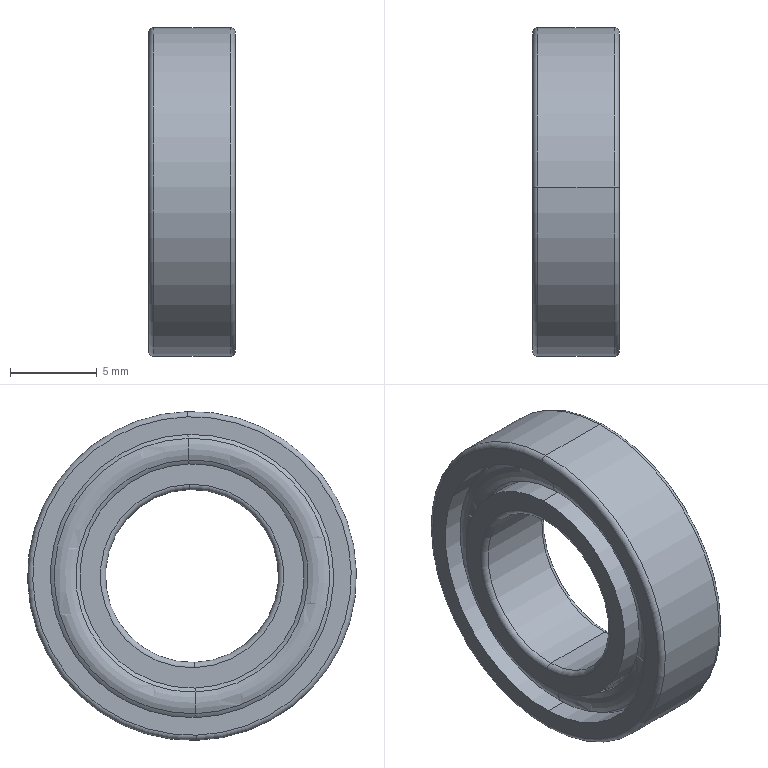Component | SolidWorks | BAR6800-3 | 1 solid | 44 faces | volume 864 mm3 | cylinder 20 | torus 20 | plane 4 | commonest cylinder face diameters 16.368 x4 15.914 x4 13.414 x4 12.96 x4 19 x2 10 x2